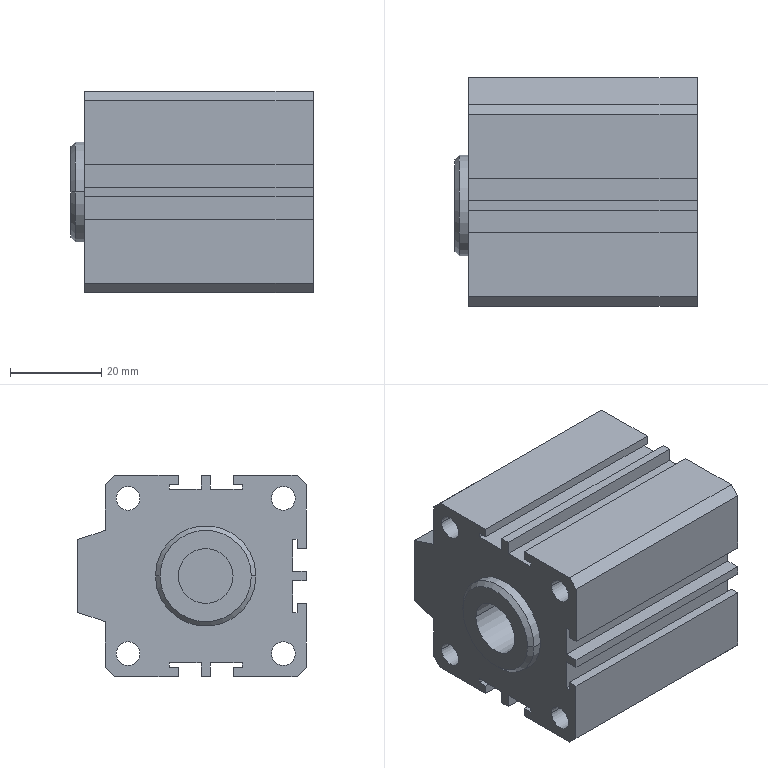Component | SolidWorks | GL9-204-_v_p_=_v-1 | 1 solid | 66 faces | box 53 x 50 x 44 mm | volume 88696 mm3 | plane 52 | cylinder 12 | cone 2 | commonest cylinder face diameters 5.2 x8 12 x2 22 x2
build123d program:
from build123d import *

# Parameters (mm, degrees)
EXTRUDE1_DEPTH = 50
SKETCH2_R      = 11
EXTRUDE2_DEPTH = 3
EXTRUDE3_DEPTH = 62.384
SKETCH4_R      = 6
EXTRUDE4_DEPTH = 43
SKETCH5_R      = 2.6
EXTRUDE5_DEPTH = 62.384
CHAMFER1_SIZE  = 1
CHAMFER2_SIZE  = 2


with BuildPart() as part:
    # Sketch1 → Extrude1 (new body)
    with BuildSketch(Plane.XY):
        Polygon((28, -8), (28, 8), (22, 10), (22, 22), (-22, 22), (-22, -22), (22, -22), (22, -10), align=None)
    extrude(amount=EXTRUDE1_DEPTH)

    # Sketch2 → Extrude2 (add)
    with BuildSketch(Plane.XY.offset(50)):
        Circle(SKETCH2_R)
    extrude(amount=EXTRUDE2_DEPTH)

    # Sketch3 → Extrude3 (cut, through all)
    with BuildSketch(Plane.XY.offset(50)):
        Polygon((-1, 19), (-8, 19), (-8, 20), (-6, 20), (-6, 22), (-1, 22), align=None)
        Polygon((-22, -1), (-19, -1), (-19, -8), (-20, -8), (-20, -6), (-22, -6), align=None)
        Polygon((1, 22), (6, 22), (6, 20), (8, 20), (8, 19), (1, 19), align=None)
        Polygon((1, -19), (8, -19), (8, -20), (6, -20), (6, -22), (1, -22), align=None)
        Polygon((-1, -22), (-6, -22), (-6, -20), (-8, -20), (-8, -19), (-1, -19), align=None)
        Polygon((-22, 6), (-22, 1), (-19, 1), (-19, 8), (-20, 8), (-20, 6), align=None)
    extrude(amount=-EXTRUDE3_DEPTH, mode=Mode.SUBTRACT)

    # Sketch4 → Extrude4 (cut)
    with BuildSketch(Plane.XY.offset(53)):
        Circle(SKETCH4_R)
    extrude(amount=-EXTRUDE4_DEPTH, mode=Mode.SUBTRACT)

    # Sketch5 → Extrude5 (cut, through all)
    with BuildSketch(Plane.XY.offset(50)):
        with Locations((17, 17)):
            Circle(SKETCH5_R)
        with Locations(Location((17, -17, 0), (0, 0, 180))):
            Circle(SKETCH5_R)
        with Locations((-17, -17)):
            Circle(SKETCH5_R)
        with Locations(Location((-17, 17, 0), (0, 0, 180))):
            Circle(SKETCH5_R)
    extrude(amount=-EXTRUDE5_DEPTH, mode=Mode.SUBTRACT)

    # Chamfer1
    chamfer1_edges = [part.edges().sort_by_distance(p)[0] for p in [
        (-11, 0, 53),
    ]]
    chamfer(chamfer1_edges, length=CHAMFER1_SIZE)

    # Chamfer2
    chamfer2_edges = [part.edges().sort_by_distance(p)[0] for p in [
        (-22, -22, 25),
        (-22, 22, 25),
        (22, 22, 25),
        (22, -22, 25),
    ]]
    chamfer(chamfer2_edges, length=CHAMFER2_SIZE)


solid = part.part

# Placed as in the assembly
solid = solid.moved(Location((65, 61.5, 0), (-90, -90, 0)))